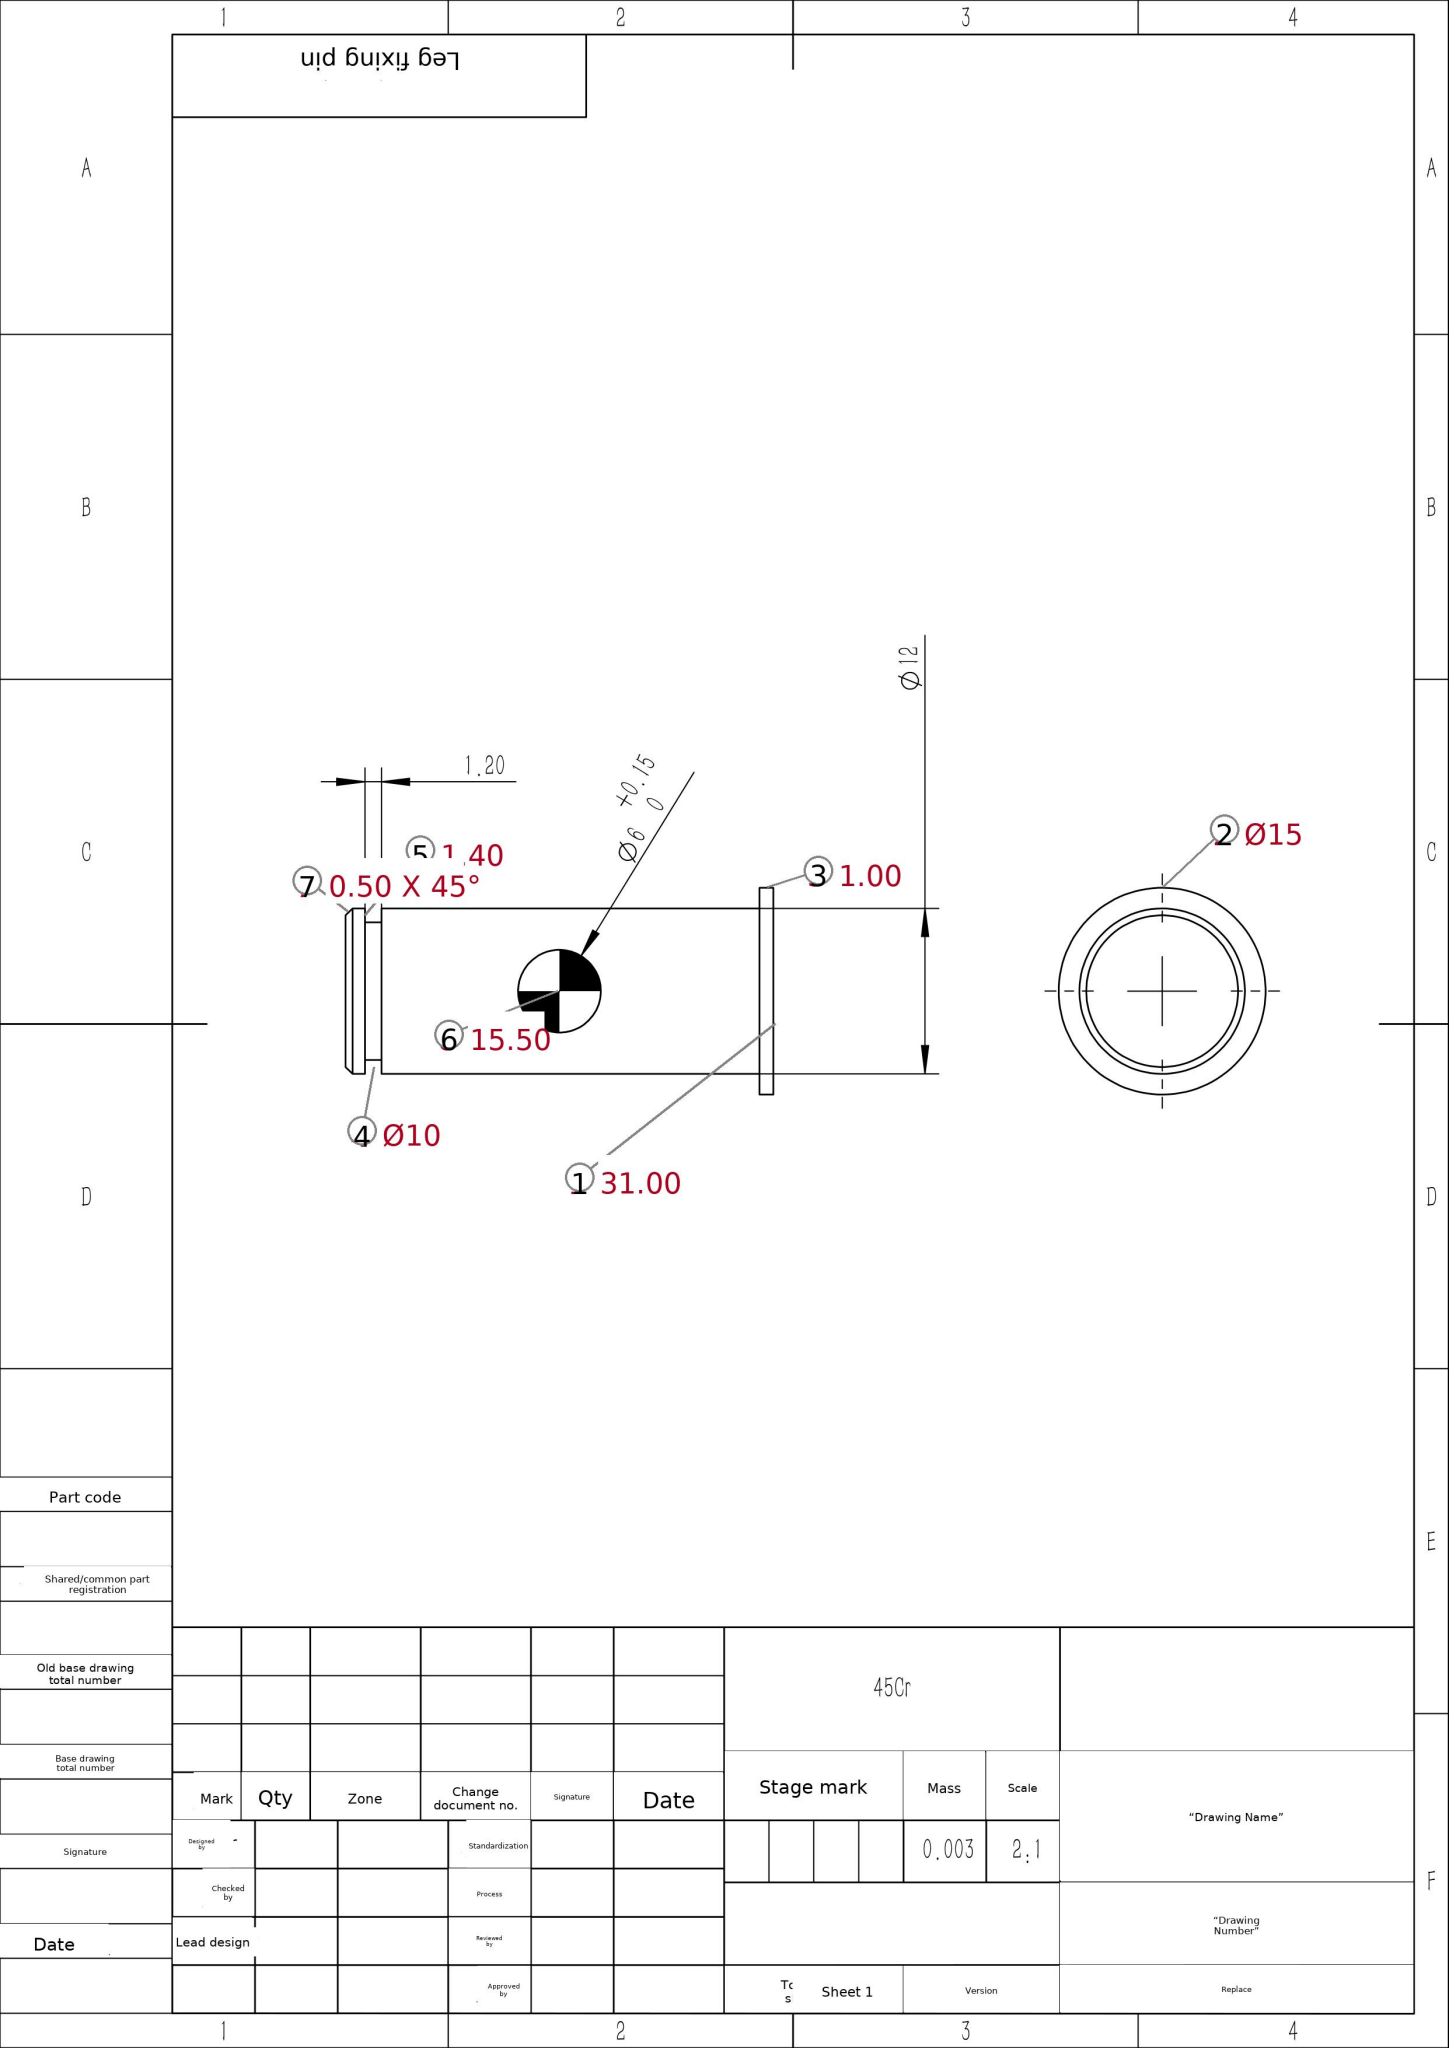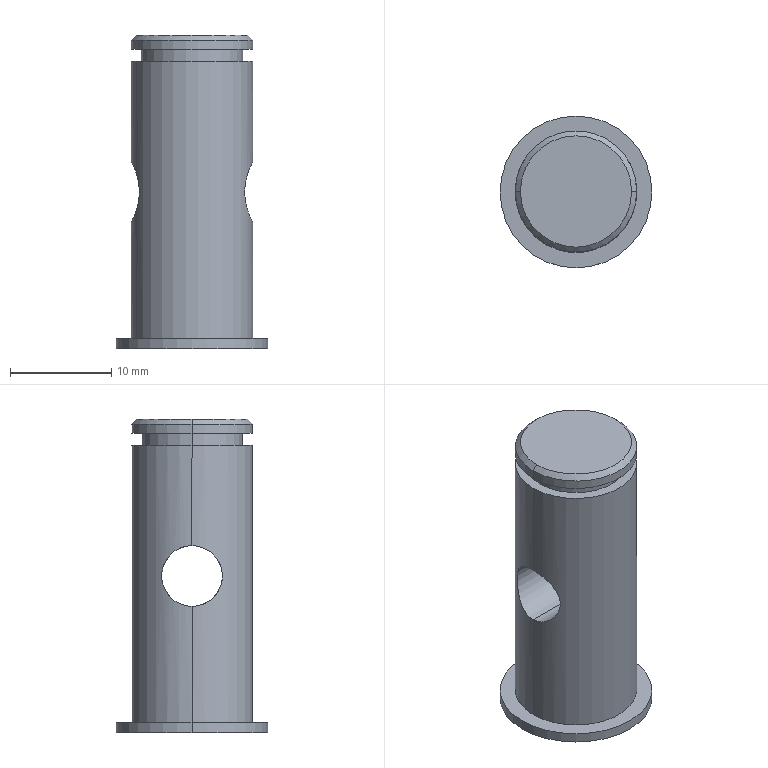Part | SolidWorks | mm | material 45Cr | 1 solid | 17 faces | box 15 x 15 x 31 mm | volume 3195 mm3 | cylinder 10 | plane 5 | cone 2 | commonest cylinder face diameters 12 x4 10 x2 15 x2 6 x2
build123d program:
from build123d import *

# Parameters (mm, degrees)
SKETCH1_R                 = 6
BOSS_EXTRUDE1_DEPTH       = 15.5
CHAMFER1_SIZE             = 0.5
SIZE_MM_DOWEL_HOLE1_D     = 6
SIZE_MM_DOWEL_HOLE1_DEPTH = 15
SIZE_MM_DOWEL_HOLE1_TIP   = 1.803
SKETCH4_R                 = 7.5
BOSS_EXTRUDE2_DEPTH       = 1
SKETCH5_W                 = 2
SKETCH5_H                 = 1.2


with BuildPart() as part:
    # Sketch1 → Boss-Extrude1 (new, symmetric)
    with BuildSketch(Plane.XY):
        Circle(SKETCH1_R)
    extrude(amount=BOSS_EXTRUDE1_DEPTH, both=True)

    # Chamfer1
    chamfer1_edges = [part.edges().sort_by_distance(p)[0] for p in [
        (-6, 0, -15.5),
        (-6, 0, 15.5),
    ]]
    chamfer(chamfer1_edges, length=CHAMFER1_SIZE)

    # Size mm Dowel Hole1
    with Locations(Plane.YZ.offset(6)):
        with Locations((0, 0)):
            Hole(SIZE_MM_DOWEL_HOLE1_D / 2, depth=SIZE_MM_DOWEL_HOLE1_DEPTH)
            with Locations((0, 0, -(SIZE_MM_DOWEL_HOLE1_DEPTH + SIZE_MM_DOWEL_HOLE1_TIP / 2))):  # 118° drill point
                Cone(0, SIZE_MM_DOWEL_HOLE1_D / 2, SIZE_MM_DOWEL_HOLE1_TIP, mode=Mode.SUBTRACT)

    # Sketch4 → Boss-Extrude2 (add)
    with BuildSketch(Plane(origin=(0, 0, -15.5), x_dir=(-1, 0, 0), z_dir=(0, 0, -1))):
        Circle(SKETCH4_R)
    extrude(amount=-BOSS_EXTRUDE2_DEPTH)

    # Sketch5 → Cut-Revolve1 (revolve, cut)
    with BuildSketch(Plane(origin=(0, 0, 0), x_dir=(1, 0, 0), z_dir=(0, 1, 0)), mode=Mode.PRIVATE) as cut_revolve1_sk:
        with Locations((6, -13.5)):
            Rectangle(SKETCH5_W, SKETCH5_H)
    revolve(cut_revolve1_sk.sketch.rotate(Axis((0, 0, 0), (0, 0, 1)), 180), axis=Axis((0, 0, 0), (0, 0, 1)), mode=Mode.SUBTRACT)


solid = part.part
STEP:
#1=CARTESIAN_POINT('',(-6.,0.,15.));
#2=VERTEX_POINT('',#1);
#3=CARTESIAN_POINT('',(6.,0.,15.));
#4=VERTEX_POINT('',#3);
#5=CARTESIAN_POINT('',(0.,0.,15.));
#6=DIRECTION('',(0.,0.,-1.));
#7=DIRECTION('',(1.,0.,0.));
#8=AXIS2_PLACEMENT_3D('',#5,#6,#7);
#9=CIRCLE('',#8,6.);
#10=EDGE_CURVE('',#2,#4,#9,.T.);
#11=ORIENTED_EDGE('',*,*,#10,.T.);
#12=CARTESIAN_POINT('',(6.,0.,14.1));
#13=VERTEX_POINT('',#12);
#14=CARTESIAN_POINT('',(6.,0.,15.5));
#15=DIRECTION('',(0.,0.,-1.));
#16=VECTOR('',#15,1000.);
#17=LINE('',#14,#16);
#18=EDGE_CURVE('',#4,#13,#17,.T.);
#19=ORIENTED_EDGE('',*,*,#18,.T.);
#20=CARTESIAN_POINT('',(-6.,0.,14.1));
#21=VERTEX_POINT('',#20);
#22=CARTESIAN_POINT('',(0.,0.,14.1));
#23=DIRECTION('',(0.,0.,-1.));
#24=DIRECTION('',(-1.,0.,0.));
#25=AXIS2_PLACEMENT_3D('',#22,#23,#24);
#26=CIRCLE('',#25,6.);
#27=EDGE_CURVE('',#21,#13,#26,.T.);
#28=ORIENTED_EDGE('',*,*,#27,.F.);
#29=CARTESIAN_POINT('',(-6.,0.,15.5));
#30=DIRECTION('',(0.,0.,-1.));
#31=VECTOR('',#30,1000.);
#32=LINE('',#29,#31);
#33=EDGE_CURVE('',#2,#21,#32,.T.);
#34=ORIENTED_EDGE('',*,*,#33,.F.);
#35=EDGE_LOOP('',(#11,#19,#28,#34));
#36=FACE_OUTER_BOUND('',#35,.T.);
#37=CARTESIAN_POINT('',(0.,0.,15.5));
#38=DIRECTION('',(0.,0.,-1.));
#39=DIRECTION('',(-1.,0.,0.));
#40=AXIS2_PLACEMENT_3D('',#37,#38,#39);
#41=CYLINDRICAL_SURFACE('',#40,6.);
#42=ADVANCED_FACE('',(#36),#41,.T.);
#43=CARTESIAN_POINT('',(5.5,0.,15.5));
#44=VERTEX_POINT('',#43);
#45=CARTESIAN_POINT('',(-5.5,0.,15.5));
#46=VERTEX_POINT('',#45);
#47=CARTESIAN_POINT('',(0.,0.,15.5));
#48=DIRECTION('',(0.,0.,1.));
#49=DIRECTION('',(1.,0.,0.));
#50=AXIS2_PLACEMENT_3D('',#47,#48,#49);
#51=CIRCLE('',#50,5.5);
#52=EDGE_CURVE('',#44,#46,#51,.T.);
#53=ORIENTED_EDGE('',*,*,#52,.F.);
#54=CARTESIAN_POINT('',(5.5,0.,15.5));
#55=DIRECTION('',(0.7071,0.,-0.7071));
#56=VECTOR('',#55,1000.);
#57=LINE('',#54,#56);
#58=EDGE_CURVE('',#44,#4,#57,.T.);
#59=ORIENTED_EDGE('',*,*,#58,.T.);
#60=ORIENTED_EDGE('',*,*,#10,.F.);
#61=CARTESIAN_POINT('',(-5.5,0.,15.5));
#62=DIRECTION('',(-0.7071,0.,-0.7071));
#63=VECTOR('',#62,1000.);
#64=LINE('',#61,#63);
#65=EDGE_CURVE('',#46,#2,#64,.T.);
#66=ORIENTED_EDGE('',*,*,#65,.F.);
#67=EDGE_LOOP('',(#53,#59,#60,#66));
#68=FACE_OUTER_BOUND('',#67,.T.);
#69=CARTESIAN_POINT('',(0.,0.,15.5));
#70=DIRECTION('',(0.,0.,-1.));
#71=DIRECTION('',(-1.,0.,0.));
#72=AXIS2_PLACEMENT_3D('',#69,#70,#71);
#73=CONICAL_SURFACE('',#72,5.5,0.7854);
#74=ADVANCED_FACE('',(#68),#73,.T.);
#75=CARTESIAN_POINT('',(-5.,0.,14.1));
#76=VERTEX_POINT('',#75);
#77=CARTESIAN_POINT('',(5.,0.,14.1));
#78=VERTEX_POINT('',#77);
#79=CARTESIAN_POINT('',(0.,0.,14.1));
#80=DIRECTION('',(0.,0.,-1.));
#81=DIRECTION('',(-1.,0.,0.));
#82=AXIS2_PLACEMENT_3D('',#79,#80,#81);
#83=CIRCLE('',#82,5.);
#84=EDGE_CURVE('',#76,#78,#83,.T.);
#85=ORIENTED_EDGE('',*,*,#84,.T.);
#86=CARTESIAN_POINT('',(5.,0.,12.9));
#87=VERTEX_POINT('',#86);
#88=CARTESIAN_POINT('',(5.,0.,0.));
#89=DIRECTION('',(0.,0.,-1.));
#90=VECTOR('',#89,1000.);
#91=LINE('',#88,#90);
#92=EDGE_CURVE('',#78,#87,#91,.T.);
#93=ORIENTED_EDGE('',*,*,#92,.T.);
#94=CARTESIAN_POINT('',(-5.,0.,12.9));
#95=VERTEX_POINT('',#94);
#96=CARTESIAN_POINT('',(0.,0.,12.9));
#97=DIRECTION('',(0.,0.,-1.));
#98=DIRECTION('',(-1.,0.,0.));
#99=AXIS2_PLACEMENT_3D('',#96,#97,#98);
#100=CIRCLE('',#99,5.);
#101=EDGE_CURVE('',#95,#87,#100,.T.);
#102=ORIENTED_EDGE('',*,*,#101,.F.);
#103=CARTESIAN_POINT('',(-5.,0.,0.));
#104=DIRECTION('',(0.,0.,-1.));
#105=VECTOR('',#104,1000.);
#106=LINE('',#103,#105);
#107=EDGE_CURVE('',#76,#95,#106,.T.);
#108=ORIENTED_EDGE('',*,*,#107,.F.);
#109=EDGE_LOOP('',(#85,#93,#102,#108));
#110=FACE_OUTER_BOUND('',#109,.T.);
#111=CARTESIAN_POINT('',(0.,0.,0.));
#112=DIRECTION('',(0.,0.,-1.));
#113=DIRECTION('',(-1.,0.,0.));
#114=AXIS2_PLACEMENT_3D('',#111,#112,#113);
#115=CYLINDRICAL_SURFACE('',#114,5.);
#116=ADVANCED_FACE('',(#110),#115,.T.);
#117=CARTESIAN_POINT('',(-7.5,0.,-14.5));
#118=VERTEX_POINT('',#117);
#119=CARTESIAN_POINT('',(7.5,0.,-14.5));
#120=VERTEX_POINT('',#119);
#121=CARTESIAN_POINT('',(0.,0.,-14.5));
#122=DIRECTION('',(0.,0.,-1.));
#123=DIRECTION('',(-1.,0.,0.));
#124=AXIS2_PLACEMENT_3D('',#121,#122,#123);
#125=CIRCLE('',#124,7.5);
#126=EDGE_CURVE('',#118,#120,#125,.T.);
#127=ORIENTED_EDGE('',*,*,#126,.T.);
#128=CARTESIAN_POINT('',(7.5,0.,-15.5));
#129=VERTEX_POINT('',#128);
#130=CARTESIAN_POINT('',(7.5,0.,-14.5));
#131=DIRECTION('',(0.,0.,-1.));
#132=VECTOR('',#131,1000.);
#133=LINE('',#130,#132);
#134=EDGE_CURVE('',#120,#129,#133,.T.);
#135=ORIENTED_EDGE('',*,*,#134,.T.);
#136=CARTESIAN_POINT('',(-7.5,0.,-15.5));
#137=VERTEX_POINT('',#136);
#138=CARTESIAN_POINT('',(0.,0.,-15.5));
#139=DIRECTION('',(0.,0.,-1.));
#140=DIRECTION('',(-1.,0.,0.));
#141=AXIS2_PLACEMENT_3D('',#138,#139,#140);
#142=CIRCLE('',#141,7.5);
#143=EDGE_CURVE('',#137,#129,#142,.T.);
#144=ORIENTED_EDGE('',*,*,#143,.F.);
#145=CARTESIAN_POINT('',(-7.5,0.,-14.5));
#146=DIRECTION('',(0.,0.,-1.));
#147=VECTOR('',#146,1000.);
#148=LINE('',#145,#147);
#149=EDGE_CURVE('',#118,#137,#148,.T.);
#150=ORIENTED_EDGE('',*,*,#149,.F.);
#151=EDGE_LOOP('',(#127,#135,#144,#150));
#152=FACE_OUTER_BOUND('',#151,.T.);
#153=CARTESIAN_POINT('',(0.,0.,-14.5));
#154=DIRECTION('',(0.,0.,-1.));
#155=DIRECTION('',(-1.,0.,0.));
#156=AXIS2_PLACEMENT_3D('',#153,#154,#155);
#157=CYLINDRICAL_SURFACE('',#156,7.5);
#158=ADVANCED_FACE('',(#152),#157,.T.);
#159=CARTESIAN_POINT('',(-6.,0.,3.));
#160=VERTEX_POINT('',#159);
#161=CARTESIAN_POINT('',(-6.,-0.,-3.));
#162=VERTEX_POINT('',#161);
#163=CARTESIAN_POINT('',(-6.,0.,3.));
#164=CARTESIAN_POINT('',(-6.,-0.2019,3.));
#165=CARTESIAN_POINT('',(-5.99,-0.3998,2.98));
#166=CARTESIAN_POINT('',(-5.951,-0.7881,2.901));
#167=CARTESIAN_POINT('',(-5.922,-0.9805,2.842));
#168=CARTESIAN_POINT('',(-5.851,-1.343,2.69));
#169=CARTESIAN_POINT('',(-5.808,-1.514,2.597));
#170=CARTESIAN_POINT('',(-5.714,-1.838,2.379));
#171=CARTESIAN_POINT('',(-5.663,-1.988,2.255));
#172=CARTESIAN_POINT('',(-5.56,-2.26,1.983));
#173=CARTESIAN_POINT('',(-5.508,-2.383,1.832));
#174=CARTESIAN_POINT('',(-5.409,-2.6,1.51));
#175=CARTESIAN_POINT('',(-5.363,-2.691,1.339));
#176=CARTESIAN_POINT('',(-5.285,-2.842,0.98));
#177=CARTESIAN_POINT('',(-5.252,-2.901,0.7881));
#178=CARTESIAN_POINT('',(-5.208,-2.98,0.3995));
#179=CARTESIAN_POINT('',(-5.196,-3.,0.2026));
#180=CARTESIAN_POINT('',(-5.196,-3.,-0.1968));
#181=CARTESIAN_POINT('',(-5.208,-2.98,-0.399));
#182=CARTESIAN_POINT('',(-5.252,-2.902,-0.7873));
#183=CARTESIAN_POINT('',(-5.284,-2.843,-0.9778));
#184=CARTESIAN_POINT('',(-5.363,-2.691,-1.341));
#185=CARTESIAN_POINT('',(-5.409,-2.598,-1.512));
#186=CARTESIAN_POINT('',(-5.508,-2.382,-1.834));
#187=CARTESIAN_POINT('',(-5.561,-2.258,-1.985));
#188=CARTESIAN_POINT('',(-5.664,-1.985,-2.257));
#189=CARTESIAN_POINT('',(-5.714,-1.837,-2.38));
#190=CARTESIAN_POINT('',(-5.809,-1.512,-2.599));
#191=CARTESIAN_POINT('',(-5.851,-1.34,-2.691));
#192=CARTESIAN_POINT('',(-5.922,-0.9795,-2.842));
#193=CARTESIAN_POINT('',(-5.951,-0.789,-2.901));
#194=CARTESIAN_POINT('',(-5.99,-0.3968,-2.98));
#195=CARTESIAN_POINT('',(-6.,-0.1992,-3.));
#196=CARTESIAN_POINT('',(-6.,-0.,-3.));
#197=B_SPLINE_CURVE_WITH_KNOTS('',3,(#163,#164,#165,#166,#167,#168,#169,#170,#171,#172,#173,#174,#175,#176,#177,#178,#179,#180,#181,#182,#183,#184,#185,#186,#187,#188,#189,#190,#191,#192,#193,#194,#195,#196),.UNSPECIFIED.,.F.,.F.,(4,2,2,2,2,2,2,2,2,2,2,2,2,2,2,2,4),(0.,0.0005964,0.001193,0.001789,0.002386,0.002982,0.003579,0.004175,0.004771,0.005368,0.005964,0.006561,0.007157,0.007754,0.00835,0.008947,0.009543),.UNSPECIFIED.);
#198=EDGE_CURVE('',#160,#162,#197,.T.);
#199=ORIENTED_EDGE('',*,*,#198,.F.);
#200=CARTESIAN_POINT('',(6.,0.,3.));
#201=VERTEX_POINT('',#200);
#202=CARTESIAN_POINT('',(6.,0.,3.));
#203=DIRECTION('',(1.,0.,0.));
#204=VECTOR('',#203,1000.);
#205=LINE('',#202,#204);
#206=EDGE_CURVE('',#160,#201,#205,.T.);
#207=ORIENTED_EDGE('',*,*,#206,.T.);
#208=CARTESIAN_POINT('',(6.,0.,-3.));
#209=VERTEX_POINT('',#208);
#210=CARTESIAN_POINT('',(6.,0.,-3.));
#211=CARTESIAN_POINT('',(6.,-0.2019,-3.));
#212=CARTESIAN_POINT('',(5.99,-0.3998,-2.98));
#213=CARTESIAN_POINT('',(5.951,-0.7881,-2.901));
#214=CARTESIAN_POINT('',(5.922,-0.9805,-2.842));
#215=CARTESIAN_POINT('',(5.851,-1.343,-2.69));
#216=CARTESIAN_POINT('',(5.808,-1.514,-2.597));
#217=CARTESIAN_POINT('',(5.714,-1.838,-2.379));
#218=CARTESIAN_POINT('',(5.663,-1.988,-2.255));
#219=CARTESIAN_POINT('',(5.56,-2.26,-1.983));
#220=CARTESIAN_POINT('',(5.508,-2.383,-1.832));
#221=CARTESIAN_POINT('',(5.409,-2.6,-1.51));
#222=CARTESIAN_POINT('',(5.363,-2.691,-1.339));
#223=CARTESIAN_POINT('',(5.285,-2.842,-0.98));
#224=CARTESIAN_POINT('',(5.252,-2.901,-0.7881));
#225=CARTESIAN_POINT('',(5.208,-2.98,-0.3995));
#226=CARTESIAN_POINT('',(5.196,-3.,-0.2026));
#227=CARTESIAN_POINT('',(5.196,-3.,0.1968));
#228=CARTESIAN_POINT('',(5.208,-2.98,0.399));
#229=CARTESIAN_POINT('',(5.252,-2.902,0.7873));
#230=CARTESIAN_POINT('',(5.284,-2.843,0.9778));
#231=CARTESIAN_POINT('',(5.363,-2.691,1.341));
#232=CARTESIAN_POINT('',(5.409,-2.598,1.512));
#233=CARTESIAN_POINT('',(5.508,-2.382,1.834));
#234=CARTESIAN_POINT('',(5.561,-2.258,1.985));
#235=CARTESIAN_POINT('',(5.664,-1.985,2.257));
#236=CARTESIAN_POINT('',(5.714,-1.837,2.38));
#237=CARTESIAN_POINT('',(5.809,-1.512,2.599));
#238=CARTESIAN_POINT('',(5.851,-1.34,2.691));
#239=CARTESIAN_POINT('',(5.922,-0.9795,2.842));
#240=CARTESIAN_POINT('',(5.951,-0.789,2.901));
#241=CARTESIAN_POINT('',(5.99,-0.3968,2.98));
#242=CARTESIAN_POINT('',(6.,-0.1992,3.));
#243=CARTESIAN_POINT('',(6.,0.,3.));
#244=B_SPLINE_CURVE_WITH_KNOTS('',3,(#210,#211,#212,#213,#214,#215,#216,#217,#218,#219,#220,#221,#222,#223,#224,#225,#226,#227,#228,#229,#230,#231,#232,#233,#234,#235,#236,#237,#238,#239,#240,#241,#242,#243),.UNSPECIFIED.,.F.,.F.,(4,2,2,2,2,2,2,2,2,2,2,2,2,2,2,2,4),(0.,0.0005964,0.001193,0.001789,0.002386,0.002982,0.003579,0.004175,0.004771,0.005368,0.005964,0.006561,0.007157,0.007754,0.00835,0.008947,0.009543),.UNSPECIFIED.);
#245=EDGE_CURVE('',#209,#201,#244,.T.);
#246=ORIENTED_EDGE('',*,*,#245,.F.);
#247=CARTESIAN_POINT('',(6.,0.,-3.));
#248=DIRECTION('',(1.,0.,0.));
#249=VECTOR('',#248,1000.);
#250=LINE('',#247,#249);
#251=EDGE_CURVE('',#162,#209,#250,.T.);
#252=ORIENTED_EDGE('',*,*,#251,.F.);
#253=EDGE_LOOP('',(#199,#207,#246,#252));
#254=FACE_OUTER_BOUND('',#253,.T.);
#255=CARTESIAN_POINT('',(6.,0.,0.));
#256=DIRECTION('',(1.,0.,0.));
#257=DIRECTION('',(0.,0.,-1.));
#258=AXIS2_PLACEMENT_3D('',#255,#256,#257);
#259=CYLINDRICAL_SURFACE('',#258,3.);
#260=ADVANCED_FACE('',(#254),#259,.F.);
#261=CARTESIAN_POINT('',(6.,0.,12.9));
#262=VERTEX_POINT('',#261);
#263=CARTESIAN_POINT('',(-6.,0.,12.9));
#264=VERTEX_POINT('',#263);
#265=CARTESIAN_POINT('',(0.,0.,12.9));
#266=DIRECTION('',(0.,0.,1.));
#267=DIRECTION('',(1.,0.,0.));
#268=AXIS2_PLACEMENT_3D('',#265,#266,#267);
#269=CIRCLE('',#268,6.);
#270=EDGE_CURVE('',#262,#264,#269,.T.);
#271=ORIENTED_EDGE('',*,*,#270,.F.);
#272=CARTESIAN_POINT('',(6.,0.,15.5));
#273=DIRECTION('',(0.,0.,-1.));
#274=VECTOR('',#273,1000.);
#275=LINE('',#272,#274);
#276=EDGE_CURVE('',#262,#201,#275,.T.);
#277=ORIENTED_EDGE('',*,*,#276,.T.);
#278=CARTESIAN_POINT('',(6.,0.,3.));
#279=CARTESIAN_POINT('',(6.,0.1988,3.));
#280=CARTESIAN_POINT('',(5.99,0.4012,2.98));
#281=CARTESIAN_POINT('',(5.951,0.79,2.901));
#282=CARTESIAN_POINT('',(5.923,0.9785,2.843));
#283=CARTESIAN_POINT('',(5.851,1.344,2.689));
#284=CARTESIAN_POINT('',(5.808,1.516,2.596));
#285=CARTESIAN_POINT('',(5.714,1.837,2.38));
#286=CARTESIAN_POINT('',(5.663,1.988,2.255));
#287=CARTESIAN_POINT('',(5.56,2.26,1.982));
#288=CARTESIAN_POINT('',(5.508,2.382,1.834));
#289=CARTESIAN_POINT('',(5.409,2.598,1.512));
#290=CARTESIAN_POINT('',(5.363,2.692,1.338));
#291=CARTESIAN_POINT('',(5.285,2.842,0.9797));
#292=CARTESIAN_POINT('',(5.253,2.9,0.7927));
#293=CARTESIAN_POINT('',(5.208,2.98,0.4013));
#294=CARTESIAN_POINT('',(5.196,3.,0.2017));
#295=CARTESIAN_POINT('',(5.196,3.,-0.1952));
#296=CARTESIAN_POINT('',(5.208,2.98,-0.3964));
#297=CARTESIAN_POINT('',(5.252,2.902,-0.7869));
#298=CARTESIAN_POINT('',(5.284,2.844,-0.9749));
#299=CARTESIAN_POINT('',(5.402,2.617,-1.519));
#300=CARTESIAN_POINT('',(5.508,2.397,-1.845));
#301=CARTESIAN_POINT('',(5.663,1.987,-2.256));
#302=CARTESIAN_POINT('',(5.714,1.838,-2.379));
#303=CARTESIAN_POINT('',(5.807,1.517,-2.595));
#304=CARTESIAN_POINT('',(5.851,1.342,-2.69));
#305=CARTESIAN_POINT('',(5.922,0.981,-2.842));
#306=CARTESIAN_POINT('',(5.951,0.7936,-2.9));
#307=CARTESIAN_POINT('',(5.99,0.4041,-2.979));
#308=CARTESIAN_POINT('',(6.,0.2015,-3.));
#309=CARTESIAN_POINT('',(6.,0.,-3.));
#310=B_SPLINE_CURVE_WITH_KNOTS('',3,(#278,#279,#280,#281,#282,#283,#284,#285,#286,#287,#288,#289,#290,#291,#292,#293,#294,#295,#296,#297,#298,#299,#300,#301,#302,#303,#304,#305,#306,#307,#308,#309),.UNSPECIFIED.,.F.,.F.,(4,2,2,2,2,2,2,2,2,2,2,2,2,2,2,4),(0.009543,0.01014,0.01073,0.01133,0.01192,0.01252,0.01312,0.01371,0.01431,0.0149,0.0155,0.01669,0.01728,0.01788,0.01847,0.01907),.UNSPECIFIED.);
#311=EDGE_CURVE('',#201,#209,#310,.T.);
#312=ORIENTED_EDGE('',*,*,#311,.T.);
#313=CARTESIAN_POINT('',(6.,0.,-14.5));
#314=VERTEX_POINT('',#313);
#315=CARTESIAN_POINT('',(6.,0.,15.5));
#316=DIRECTION('',(0.,0.,-1.));
#317=VECTOR('',#316,1000.);
#318=LINE('',#315,#317);
#319=EDGE_CURVE('',#209,#314,#318,.T.);
#320=ORIENTED_EDGE('',*,*,#319,.T.);
#321=CARTESIAN_POINT('',(-6.,0.,-14.5));
#322=VERTEX_POINT('',#321);
#323=CARTESIAN_POINT('',(0.,0.,-14.5));
#324=DIRECTION('',(0.,0.,-1.));
#325=DIRECTION('',(-1.,0.,0.));
#326=AXIS2_PLACEMENT_3D('',#323,#324,#325);
#327=CIRCLE('',#326,6.);
#328=EDGE_CURVE('',#322,#314,#327,.T.);
#329=ORIENTED_EDGE('',*,*,#328,.F.);
#330=CARTESIAN_POINT('',(-6.,0.,15.5));
#331=DIRECTION('',(0.,0.,-1.));
#332=VECTOR('',#331,1000.);
#333=LINE('',#330,#332);
#334=EDGE_CURVE('',#162,#322,#333,.T.);
#335=ORIENTED_EDGE('',*,*,#334,.F.);
#336=CARTESIAN_POINT('',(-6.,-0.,-3.));
#337=CARTESIAN_POINT('',(-6.,0.1988,-3.));
#338=CARTESIAN_POINT('',(-5.99,0.4012,-2.98));
#339=CARTESIAN_POINT('',(-5.951,0.79,-2.901));
#340=CARTESIAN_POINT('',(-5.923,0.9785,-2.843));
#341=CARTESIAN_POINT('',(-5.851,1.344,-2.689));
#342=CARTESIAN_POINT('',(-5.808,1.516,-2.596));
#343=CARTESIAN_POINT('',(-5.714,1.837,-2.38));
#344=CARTESIAN_POINT('',(-5.663,1.988,-2.255));
#345=CARTESIAN_POINT('',(-5.56,2.26,-1.982));
#346=CARTESIAN_POINT('',(-5.508,2.382,-1.834));
#347=CARTESIAN_POINT('',(-5.409,2.598,-1.512));
#348=CARTESIAN_POINT('',(-5.363,2.692,-1.338));
#349=CARTESIAN_POINT('',(-5.285,2.842,-0.9797));
#350=CARTESIAN_POINT('',(-5.253,2.9,-0.7927));
#351=CARTESIAN_POINT('',(-5.208,2.98,-0.4013));
#352=CARTESIAN_POINT('',(-5.196,3.,-0.2017));
#353=CARTESIAN_POINT('',(-5.196,3.,0.1952));
#354=CARTESIAN_POINT('',(-5.208,2.98,0.3964));
#355=CARTESIAN_POINT('',(-5.252,2.902,0.7869));
#356=CARTESIAN_POINT('',(-5.284,2.844,0.9749));
#357=CARTESIAN_POINT('',(-5.402,2.617,1.519));
#358=CARTESIAN_POINT('',(-5.508,2.397,1.845));
#359=CARTESIAN_POINT('',(-5.663,1.987,2.256));
#360=CARTESIAN_POINT('',(-5.714,1.838,2.379));
#361=CARTESIAN_POINT('',(-5.807,1.517,2.595));
#362=CARTESIAN_POINT('',(-5.851,1.342,2.69));
#363=CARTESIAN_POINT('',(-5.922,0.981,2.842));
#364=CARTESIAN_POINT('',(-5.951,0.7936,2.9));
#365=CARTESIAN_POINT('',(-5.99,0.4041,2.979));
#366=CARTESIAN_POINT('',(-6.,0.2015,3.));
#367=CARTESIAN_POINT('',(-6.,0.,3.));
#368=B_SPLINE_CURVE_WITH_KNOTS('',3,(#336,#337,#338,#339,#340,#341,#342,#343,#344,#345,#346,#347,#348,#349,#350,#351,#352,#353,#354,#355,#356,#357,#358,#359,#360,#361,#362,#363,#364,#365,#366,#367),.UNSPECIFIED.,.F.,.F.,(4,2,2,2,2,2,2,2,2,2,2,2,2,2,2,4),(0.009543,0.01014,0.01073,0.01133,0.01192,0.01252,0.01312,0.01371,0.01431,0.0149,0.0155,0.01669,0.01728,0.01788,0.01847,0.01907),.UNSPECIFIED.);
#369=EDGE_CURVE('',#162,#160,#368,.T.);
#370=ORIENTED_EDGE('',*,*,#369,.T.);
#371=CARTESIAN_POINT('',(-6.,0.,15.5));
#372=DIRECTION('',(0.,0.,-1.));
#373=VECTOR('',#372,1000.);
#374=LINE('',#371,#373);
#375=EDGE_CURVE('',#264,#160,#374,.T.);
#376=ORIENTED_EDGE('',*,*,#375,.F.);
#377=EDGE_LOOP('',(#271,#277,#312,#320,#329,#335,#370,#376));
#378=FACE_OUTER_BOUND('',#377,.T.);
#379=CARTESIAN_POINT('',(0.,0.,15.5));
#380=DIRECTION('',(0.,0.,-1.));
#381=DIRECTION('',(-1.,0.,0.));
#382=AXIS2_PLACEMENT_3D('',#379,#380,#381);
#383=CYLINDRICAL_SURFACE('',#382,6.);
#384=ADVANCED_FACE('',(#378),#383,.T.);
#385=ORIENTED_EDGE('',*,*,#276,.F.);
#386=CARTESIAN_POINT('',(0.,0.,12.9));
#387=DIRECTION('',(0.,0.,1.));
#388=DIRECTION('',(1.,0.,0.));
#389=AXIS2_PLACEMENT_3D('',#386,#387,#388);
#390=CIRCLE('',#389,6.);
#391=EDGE_CURVE('',#264,#262,#390,.T.);
#392=ORIENTED_EDGE('',*,*,#391,.F.);
#393=ORIENTED_EDGE('',*,*,#375,.T.);
#394=ORIENTED_EDGE('',*,*,#198,.T.);
#395=ORIENTED_EDGE('',*,*,#334,.T.);
#396=CARTESIAN_POINT('',(0.,0.,-14.5));
#397=DIRECTION('',(0.,0.,-1.));
#398=DIRECTION('',(-1.,0.,0.));
#399=AXIS2_PLACEMENT_3D('',#396,#397,#398);
#400=CIRCLE('',#399,6.);
#401=EDGE_CURVE('',#314,#322,#400,.T.);
#402=ORIENTED_EDGE('',*,*,#401,.F.);
#403=ORIENTED_EDGE('',*,*,#319,.F.);
#404=ORIENTED_EDGE('',*,*,#245,.T.);
#405=EDGE_LOOP('',(#385,#392,#393,#394,#395,#402,#403,#404));
#406=FACE_OUTER_BOUND('',#405,.T.);
#407=CARTESIAN_POINT('',(0.,0.,15.5));
#408=DIRECTION('',(0.,0.,-1.));
#409=DIRECTION('',(-1.,0.,0.));
#410=AXIS2_PLACEMENT_3D('',#407,#408,#409);
#411=CYLINDRICAL_SURFACE('',#410,6.);
#412=ADVANCED_FACE('',(#406),#411,.T.);
#413=ORIENTED_EDGE('',*,*,#206,.F.);
#414=ORIENTED_EDGE('',*,*,#369,.F.);
#415=ORIENTED_EDGE('',*,*,#251,.T.);
#416=ORIENTED_EDGE('',*,*,#311,.F.);
#417=EDGE_LOOP('',(#413,#414,#415,#416));
#418=FACE_OUTER_BOUND('',#417,.T.);
#419=CARTESIAN_POINT('',(6.,0.,0.));
#420=DIRECTION('',(1.,0.,0.));
#421=DIRECTION('',(0.,0.,-1.));
#422=AXIS2_PLACEMENT_3D('',#419,#420,#421);
#423=CYLINDRICAL_SURFACE('',#422,3.);
#424=ADVANCED_FACE('',(#418),#423,.F.);
#425=ORIENTED_EDGE('',*,*,#134,.F.);
#426=CARTESIAN_POINT('',(0.,0.,-14.5));
#427=DIRECTION('',(0.,0.,-1.));
#428=DIRECTION('',(-1.,0.,0.));
#429=AXIS2_PLACEMENT_3D('',#426,#427,#428);
#430=CIRCLE('',#429,7.5);
#431=EDGE_CURVE('',#120,#118,#430,.T.);
#432=ORIENTED_EDGE('',*,*,#431,.T.);
#433=ORIENTED_EDGE('',*,*,#149,.T.);
#434=CARTESIAN_POINT('',(0.,0.,-15.5));
#435=DIRECTION('',(0.,0.,-1.));
#436=DIRECTION('',(-1.,0.,0.));
#437=AXIS2_PLACEMENT_3D('',#434,#435,#436);
#438=CIRCLE('',#437,7.5);
#439=EDGE_CURVE('',#129,#137,#438,.T.);
#440=ORIENTED_EDGE('',*,*,#439,.F.);
#441=EDGE_LOOP('',(#425,#432,#433,#440));
#442=FACE_OUTER_BOUND('',#441,.T.);
#443=CARTESIAN_POINT('',(0.,0.,-14.5));
#444=DIRECTION('',(0.,0.,-1.));
#445=DIRECTION('',(-1.,0.,0.));
#446=AXIS2_PLACEMENT_3D('',#443,#444,#445);
#447=CYLINDRICAL_SURFACE('',#446,7.5);
#448=ADVANCED_FACE('',(#442),#447,.T.);
#449=ORIENTED_EDGE('',*,*,#328,.T.);
#450=ORIENTED_EDGE('',*,*,#401,.T.);
#451=EDGE_LOOP('',(#449,#450));
#452=FACE_BOUND('',#451,.T.);
#453=ORIENTED_EDGE('',*,*,#126,.F.);
#454=ORIENTED_EDGE('',*,*,#431,.F.);
#455=EDGE_LOOP('',(#453,#454));
#456=FACE_OUTER_BOUND('',#455,.T.);
#457=CARTESIAN_POINT('',(0.,0.,-14.5));
#458=DIRECTION('',(0.,0.,-1.));
#459=DIRECTION('',(-1.,0.,0.));
#460=AXIS2_PLACEMENT_3D('',#457,#458,#459);
#461=PLANE('',#460);
#462=ADVANCED_FACE('',(#452,#456),#461,.F.);
#463=ORIENTED_EDGE('',*,*,#143,.T.);
#464=ORIENTED_EDGE('',*,*,#439,.T.);
#465=EDGE_LOOP('',(#463,#464));
#466=FACE_OUTER_BOUND('',#465,.T.);
#467=CARTESIAN_POINT('',(0.,0.,-15.5));
#468=DIRECTION('',(0.,0.,1.));
#469=DIRECTION('',(1.,0.,0.));
#470=AXIS2_PLACEMENT_3D('',#467,#468,#469);
#471=PLANE('',#470);
#472=ADVANCED_FACE('',(#466),#471,.F.);
#473=ORIENTED_EDGE('',*,*,#84,.F.);
#474=CARTESIAN_POINT('',(0.,0.,14.1));
#475=DIRECTION('',(0.,0.,-1.));
#476=DIRECTION('',(-1.,0.,0.));
#477=AXIS2_PLACEMENT_3D('',#474,#475,#476);
#478=CIRCLE('',#477,5.);
#479=EDGE_CURVE('',#78,#76,#478,.T.);
#480=ORIENTED_EDGE('',*,*,#479,.F.);
#481=EDGE_LOOP('',(#473,#480));
#482=FACE_BOUND('',#481,.T.);
#483=ORIENTED_EDGE('',*,*,#27,.T.);
#484=CARTESIAN_POINT('',(0.,0.,14.1));
#485=DIRECTION('',(0.,0.,-1.));
#486=DIRECTION('',(-1.,0.,0.));
#487=AXIS2_PLACEMENT_3D('',#484,#485,#486);
#488=CIRCLE('',#487,6.);
#489=EDGE_CURVE('',#13,#21,#488,.T.);
#490=ORIENTED_EDGE('',*,*,#489,.T.);
#491=EDGE_LOOP('',(#483,#490));
#492=FACE_OUTER_BOUND('',#491,.T.);
#493=CARTESIAN_POINT('',(7.,0.,14.1));
#494=DIRECTION('',(0.,0.,-1.));
#495=DIRECTION('',(-1.,0.,0.));
#496=AXIS2_PLACEMENT_3D('',#493,#494,#495);
#497=PLANE('',#496);
#498=ADVANCED_FACE('',(#482,#492),#497,.T.);
#499=ORIENTED_EDGE('',*,*,#101,.T.);
#500=CARTESIAN_POINT('',(0.,0.,12.9));
#501=DIRECTION('',(0.,0.,-1.));
#502=DIRECTION('',(-1.,0.,0.));
#503=AXIS2_PLACEMENT_3D('',#500,#501,#502);
#504=CIRCLE('',#503,5.);
#505=EDGE_CURVE('',#87,#95,#504,.T.);
#506=ORIENTED_EDGE('',*,*,#505,.T.);
#507=EDGE_LOOP('',(#499,#506));
#508=FACE_BOUND('',#507,.T.);
#509=ORIENTED_EDGE('',*,*,#391,.T.);
#510=ORIENTED_EDGE('',*,*,#270,.T.);
#511=EDGE_LOOP('',(#509,#510));
#512=FACE_OUTER_BOUND('',#511,.T.);
#513=CARTESIAN_POINT('',(7.,0.,12.9));
#514=DIRECTION('',(0.,0.,1.));
#515=DIRECTION('',(1.,0.,0.));
#516=AXIS2_PLACEMENT_3D('',#513,#514,#515);
#517=PLANE('',#516);
#518=ADVANCED_FACE('',(#508,#512),#517,.T.);
#519=ORIENTED_EDGE('',*,*,#92,.F.);
#520=ORIENTED_EDGE('',*,*,#479,.T.);
#521=ORIENTED_EDGE('',*,*,#107,.T.);
#522=ORIENTED_EDGE('',*,*,#505,.F.);
#523=EDGE_LOOP('',(#519,#520,#521,#522));
#524=FACE_OUTER_BOUND('',#523,.T.);
#525=CARTESIAN_POINT('',(0.,0.,0.));
#526=DIRECTION('',(0.,0.,-1.));
#527=DIRECTION('',(-1.,0.,0.));
#528=AXIS2_PLACEMENT_3D('',#525,#526,#527);
#529=CYLINDRICAL_SURFACE('',#528,5.);
#530=ADVANCED_FACE('',(#524),#529,.T.);
#531=CARTESIAN_POINT('',(0.,0.,15.5));
#532=DIRECTION('',(0.,0.,1.));
#533=DIRECTION('',(1.,0.,0.));
#534=AXIS2_PLACEMENT_3D('',#531,#532,#533);
#535=CIRCLE('',#534,5.5);
#536=EDGE_CURVE('',#46,#44,#535,.T.);
#537=ORIENTED_EDGE('',*,*,#536,.T.);
#538=ORIENTED_EDGE('',*,*,#52,.T.);
#539=EDGE_LOOP('',(#537,#538));
#540=FACE_OUTER_BOUND('',#539,.T.);
#541=CARTESIAN_POINT('',(0.,0.,15.5));
#542=DIRECTION('',(0.,0.,1.));
#543=DIRECTION('',(1.,0.,0.));
#544=AXIS2_PLACEMENT_3D('',#541,#542,#543);
#545=PLANE('',#544);
#546=ADVANCED_FACE('',(#540),#545,.T.);
#547=ORIENTED_EDGE('',*,*,#58,.F.);
#548=ORIENTED_EDGE('',*,*,#536,.F.);
#549=ORIENTED_EDGE('',*,*,#65,.T.);
#550=CARTESIAN_POINT('',(0.,0.,15.));
#551=DIRECTION('',(0.,0.,-1.));
#552=DIRECTION('',(1.,0.,0.));
#553=AXIS2_PLACEMENT_3D('',#550,#551,#552);
#554=CIRCLE('',#553,6.);
#555=EDGE_CURVE('',#4,#2,#554,.T.);
#556=ORIENTED_EDGE('',*,*,#555,.F.);
#557=EDGE_LOOP('',(#547,#548,#549,#556));
#558=FACE_OUTER_BOUND('',#557,.T.);
#559=CARTESIAN_POINT('',(0.,0.,15.5));
#560=DIRECTION('',(0.,0.,-1.));
#561=DIRECTION('',(-1.,0.,0.));
#562=AXIS2_PLACEMENT_3D('',#559,#560,#561);
#563=CONICAL_SURFACE('',#562,5.5,0.7854);
#564=ADVANCED_FACE('',(#558),#563,.T.);
#565=ORIENTED_EDGE('',*,*,#18,.F.);
#566=ORIENTED_EDGE('',*,*,#555,.T.);
#567=ORIENTED_EDGE('',*,*,#33,.T.);
#568=ORIENTED_EDGE('',*,*,#489,.F.);
#569=EDGE_LOOP('',(#565,#566,#567,#568));
#570=FACE_OUTER_BOUND('',#569,.T.);
#571=CARTESIAN_POINT('',(0.,0.,15.5));
#572=DIRECTION('',(0.,0.,-1.));
#573=DIRECTION('',(-1.,0.,0.));
#574=AXIS2_PLACEMENT_3D('',#571,#572,#573);
#575=CYLINDRICAL_SURFACE('',#574,6.);
#576=ADVANCED_FACE('',(#570),#575,.T.);
#577=CLOSED_SHELL('',(#42,#74,#116,#158,#260,#384,#412,#424,#448,#462,#472,#498,#518,#530,#546,#564,#576));
#578=MANIFOLD_SOLID_BREP('',#577);
#579=CARTESIAN_POINT('',(0.,0.,0.));
#580=DIRECTION('',(0.,0.,1.));
#581=DIRECTION('',(1.,0.,0.));
#582=AXIS2_PLACEMENT_3D('',#579,#580,#581);
#583=(LENGTH_UNIT()NAMED_UNIT(*)SI_UNIT(.MILLI.,.METRE.));
#584=UNCERTAINTY_MEASURE_WITH_UNIT(LENGTH_MEASURE(0.00001),#583,'','');
#585=(NAMED_UNIT(*)PLANE_ANGLE_UNIT()SI_UNIT($,.RADIAN.));
#586=(NAMED_UNIT(*)SI_UNIT($,.STERADIAN.)SOLID_ANGLE_UNIT());
#587=(GEOMETRIC_REPRESENTATION_CONTEXT(3)GLOBAL_UNCERTAINTY_ASSIGNED_CONTEXT((#584))GLOBAL_UNIT_ASSIGNED_CONTEXT((#583,#585,#586))REPRESENTATION_CONTEXT('',''));
#588=ADVANCED_BREP_SHAPE_REPRESENTATION('',(#578,#582),#587);